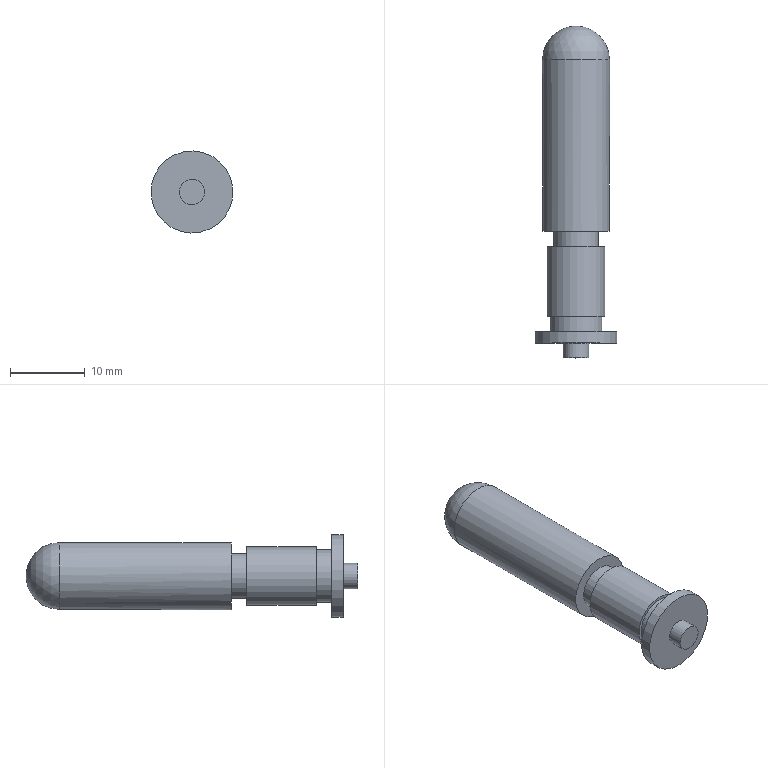Component | NX | VALVE_CORE | 1 solid | 13 faces | box 11 x 44.5 x 11 mm | volume 2399 mm3 | cylinder 6 | plane 6 | sphere 1 | commonest cylinder face diameters 11 x1 3.4 x1 7 x1 7.8 x1 6 x1 9 x1
STEP:
#1=CARTESIAN_POINT('',(0.,0.,0.));
#2=DIRECTION('',(0.,0.,1.));
#3=DIRECTION('',(1.,0.,0.));
#4=AXIS2_PLACEMENT_3D('',#1,#2,#3);
#5=CARTESIAN_POINT('',(9.389,-116.169,-3.008));
#6=VERTEX_POINT('',#5);
#7=CARTESIAN_POINT('',(13.994,-116.169,-0.));
#8=DIRECTION('',(0.,1.,0.));
#9=DIRECTION('',(-0.8372,0.,-0.5469));
#10=AXIS2_PLACEMENT_3D('',#7,#8,#9);
#11=CIRCLE('',#10,5.5);
#12=CARTESIAN_POINT('',(13.994,-116.169,-0.));
#13=DIRECTION('',(0.,-1.,0.));
#14=DIRECTION('',(-0.5469,0.,0.8372));
#15=AXIS2_PLACEMENT_3D('',#12,#13,#14);
#16=CYLINDRICAL_SURFACE('',#15,5.5);
#17=CARTESIAN_POINT('',(7.854,0.));
#18=DIRECTION('',(-1.,0.));
#19=VECTOR('',#18,1.);
#20=LINE('',#17,#19);
#21=(GEOMETRIC_REPRESENTATION_CONTEXT(2)PARAMETRIC_REPRESENTATION_CONTEXT()REPRESENTATION_CONTEXT('',''));
#22=DEFINITIONAL_REPRESENTATION('',(#20),#21);
#23=PCURVE('',#16,#22);
#24=CARTESIAN_POINT('',(13.994,-116.169,-0.));
#25=DIRECTION('',(0.,1.,0.));
#26=DIRECTION('',(0.5469,0.,-0.8372));
#27=AXIS2_PLACEMENT_3D('',#24,#25,#26);
#28=PLANE('',#27);
#29=CARTESIAN_POINT('',(0.,0.));
#30=DIRECTION('',(0.,1.));
#31=AXIS2_PLACEMENT_2D('',#29,#30);
#32=CIRCLE('',#31,5.5);
#33=(GEOMETRIC_REPRESENTATION_CONTEXT(2)PARAMETRIC_REPRESENTATION_CONTEXT()REPRESENTATION_CONTEXT('',''));
#34=DEFINITIONAL_REPRESENTATION('',(#32),#33);
#35=PCURVE('',#28,#34);
#36=SURFACE_CURVE('',#11,(#23,#35),.PCURVE_S1.);
#37=EDGE_CURVE('',#6,#6,#36,.T.);
#38=ORIENTED_EDGE('',*,*,#37,.F.);
#39=CARTESIAN_POINT('',(9.389,-117.669,-3.008));
#40=VERTEX_POINT('',#39);
#41=CARTESIAN_POINT('',(9.389,-116.169,-3.008));
#42=CARTESIAN_POINT('',(9.389,-117.669,-3.008));
#43=B_SPLINE_CURVE_WITH_KNOTS('',1,(#41,#42),.UNSPECIFIED.,.F.,.F.,(2,2),(0.,1.5),.PIECEWISE_BEZIER_KNOTS.);
#44=CARTESIAN_POINT('',(7.854,0.));
#45=DIRECTION('',(0.,1.));
#46=VECTOR('',#45,1.);
#47=LINE('',#44,#46);
#48=(GEOMETRIC_REPRESENTATION_CONTEXT(2)PARAMETRIC_REPRESENTATION_CONTEXT()REPRESENTATION_CONTEXT('',''));
#49=DEFINITIONAL_REPRESENTATION('',(#47),#48);
#50=PCURVE('',#16,#49);
#51=CARTESIAN_POINT('',(1.571,0.));
#52=DIRECTION('',(0.,1.));
#53=VECTOR('',#52,1.);
#54=LINE('',#51,#53);
#55=(GEOMETRIC_REPRESENTATION_CONTEXT(2)PARAMETRIC_REPRESENTATION_CONTEXT()REPRESENTATION_CONTEXT('',''));
#56=DEFINITIONAL_REPRESENTATION('',(#54),#55);
#57=PCURVE('',#16,#56);
#58=SEAM_CURVE('',#43,(#50,#57),.PCURVE_S1.);
#59=EDGE_CURVE('',#6,#40,#58,.T.);
#60=ORIENTED_EDGE('',*,*,#59,.T.);
#61=CARTESIAN_POINT('',(13.994,-117.669,-0.));
#62=DIRECTION('',(0.,1.,0.));
#63=DIRECTION('',(-0.8372,0.,-0.5469));
#64=AXIS2_PLACEMENT_3D('',#61,#62,#63);
#65=CIRCLE('',#64,5.5);
#66=CARTESIAN_POINT('',(7.854,1.5));
#67=DIRECTION('',(-1.,0.));
#68=VECTOR('',#67,1.);
#69=LINE('',#66,#68);
#70=(GEOMETRIC_REPRESENTATION_CONTEXT(2)PARAMETRIC_REPRESENTATION_CONTEXT()REPRESENTATION_CONTEXT('',''));
#71=DEFINITIONAL_REPRESENTATION('',(#69),#70);
#72=PCURVE('',#16,#71);
#73=CARTESIAN_POINT('',(13.994,-117.669,-0.));
#74=DIRECTION('',(0.,1.,0.));
#75=DIRECTION('',(0.5469,0.,-0.8372));
#76=AXIS2_PLACEMENT_3D('',#73,#74,#75);
#77=PLANE('',#76);
#78=CARTESIAN_POINT('',(0.,0.));
#79=DIRECTION('',(0.,1.));
#80=AXIS2_PLACEMENT_2D('',#78,#79);
#81=CIRCLE('',#80,5.5);
#82=(GEOMETRIC_REPRESENTATION_CONTEXT(2)PARAMETRIC_REPRESENTATION_CONTEXT()REPRESENTATION_CONTEXT('',''));
#83=DEFINITIONAL_REPRESENTATION('',(#81),#82);
#84=PCURVE('',#77,#83);
#85=SURFACE_CURVE('',#65,(#72,#84),.PCURVE_S1.);
#86=EDGE_CURVE('',#40,#40,#85,.T.);
#87=ORIENTED_EDGE('',*,*,#86,.T.);
#88=ORIENTED_EDGE('',*,*,#59,.F.);
#89=EDGE_LOOP('',(#38,#60,#87,#88));
#90=FACE_BOUND('',#89,.T.);
#91=ADVANCED_FACE('',(#90),#16,.T.);
#92=CARTESIAN_POINT('',(11.064,-116.169,-1.914));
#93=VERTEX_POINT('',#92);
#94=CARTESIAN_POINT('',(13.994,-116.169,-0.));
#95=DIRECTION('',(0.,1.,0.));
#96=DIRECTION('',(-0.8372,0.,-0.5469));
#97=AXIS2_PLACEMENT_3D('',#94,#95,#96);
#98=CIRCLE('',#97,3.5);
#99=CARTESIAN_POINT('',(0.,0.));
#100=DIRECTION('',(0.,1.));
#101=AXIS2_PLACEMENT_2D('',#99,#100);
#102=CIRCLE('',#101,3.5);
#103=(GEOMETRIC_REPRESENTATION_CONTEXT(2)PARAMETRIC_REPRESENTATION_CONTEXT()REPRESENTATION_CONTEXT('',''));
#104=DEFINITIONAL_REPRESENTATION('',(#102),#103);
#105=PCURVE('',#28,#104);
#106=CARTESIAN_POINT('',(13.994,-114.069,-0.));
#107=DIRECTION('',(0.,-1.,0.));
#108=DIRECTION('',(-0.5469,0.,0.8372));
#109=AXIS2_PLACEMENT_3D('',#106,#107,#108);
#110=CYLINDRICAL_SURFACE('',#109,3.5);
#111=CARTESIAN_POINT('',(7.854,2.1));
#112=DIRECTION('',(-1.,0.));
#113=VECTOR('',#112,1.);
#114=LINE('',#111,#113);
#115=(GEOMETRIC_REPRESENTATION_CONTEXT(2)PARAMETRIC_REPRESENTATION_CONTEXT()REPRESENTATION_CONTEXT('',''));
#116=DEFINITIONAL_REPRESENTATION('',(#114),#115);
#117=PCURVE('',#110,#116);
#118=SURFACE_CURVE('',#98,(#105,#117),.PCURVE_S1.);
#119=EDGE_CURVE('',#93,#93,#118,.T.);
#120=ORIENTED_EDGE('',*,*,#119,.F.);
#121=EDGE_LOOP('',(#120));
#122=FACE_BOUND('',#121,.T.);
#123=ORIENTED_EDGE('',*,*,#37,.T.);
#124=EDGE_LOOP('',(#123));
#125=FACE_BOUND('',#124,.T.);
#126=ADVANCED_FACE('',(#122,#125),#28,.T.);
#127=CARTESIAN_POINT('',(12.571,-117.669,-0.9298));
#128=VERTEX_POINT('',#127);
#129=CARTESIAN_POINT('',(13.994,-117.669,-0.));
#130=DIRECTION('',(0.,-1.,0.));
#131=DIRECTION('',(-0.8372,0.,-0.5469));
#132=AXIS2_PLACEMENT_3D('',#129,#130,#131);
#133=CIRCLE('',#132,1.7);
#134=CARTESIAN_POINT('',(0.,1.7));
#135=CARTESIAN_POINT('',(2.944,1.7));
#136=CARTESIAN_POINT('',(1.472,-0.85));
#137=CARTESIAN_POINT('',(0.,-3.4));
#138=CARTESIAN_POINT('',(-1.472,-0.85));
#139=CARTESIAN_POINT('',(-2.944,1.7));
#140=CARTESIAN_POINT('',(0.,1.7));
#141=(BOUNDED_CURVE()B_SPLINE_CURVE(2,(#134,#135,#136,#137,#138,#139,#140),.UNSPECIFIED.,.T.,.F.)B_SPLINE_CURVE_WITH_KNOTS((1,2,2,2,2,1),(-2.094,0.,2.094,4.189,6.283,8.378),.UNSPECIFIED.)CURVE()GEOMETRIC_REPRESENTATION_ITEM()RATIONAL_B_SPLINE_CURVE((1.,0.5,1.,0.5,1.,0.5,1.))REPRESENTATION_ITEM(''));
#142=(GEOMETRIC_REPRESENTATION_CONTEXT(2)PARAMETRIC_REPRESENTATION_CONTEXT()REPRESENTATION_CONTEXT('',''));
#143=DEFINITIONAL_REPRESENTATION('',(#141),#142);
#144=PCURVE('',#77,#143);
#145=CARTESIAN_POINT('',(13.994,-119.669,-0.));
#146=DIRECTION('',(0.,1.,0.));
#147=DIRECTION('',(0.5469,0.,-0.8372));
#148=AXIS2_PLACEMENT_3D('',#145,#146,#147);
#149=CYLINDRICAL_SURFACE('',#148,1.7);
#150=CARTESIAN_POINT('',(7.854,2.));
#151=DIRECTION('',(-1.,0.));
#152=VECTOR('',#151,1.);
#153=LINE('',#150,#152);
#154=(GEOMETRIC_REPRESENTATION_CONTEXT(2)PARAMETRIC_REPRESENTATION_CONTEXT()REPRESENTATION_CONTEXT('',''));
#155=DEFINITIONAL_REPRESENTATION('',(#153),#154);
#156=PCURVE('',#149,#155);
#157=SURFACE_CURVE('',#133,(#144,#156),.PCURVE_S1.);
#158=EDGE_CURVE('',#128,#128,#157,.T.);
#159=ORIENTED_EDGE('',*,*,#158,.F.);
#160=EDGE_LOOP('',(#159));
#161=FACE_BOUND('',#160,.T.);
#162=ORIENTED_EDGE('',*,*,#86,.F.);
#163=EDGE_LOOP('',(#162));
#164=FACE_BOUND('',#163,.T.);
#165=ADVANCED_FACE('',(#161,#164),#77,.F.);
#166=CARTESIAN_POINT('',(12.571,-119.669,-0.9298));
#167=VERTEX_POINT('',#166);
#168=CARTESIAN_POINT('',(13.994,-119.669,-0.));
#169=DIRECTION('',(0.,-1.,0.));
#170=DIRECTION('',(-0.8372,0.,-0.5469));
#171=AXIS2_PLACEMENT_3D('',#168,#169,#170);
#172=CIRCLE('',#171,1.7);
#173=CARTESIAN_POINT('',(7.854,0.));
#174=DIRECTION('',(-1.,0.));
#175=VECTOR('',#174,1.);
#176=LINE('',#173,#175);
#177=(GEOMETRIC_REPRESENTATION_CONTEXT(2)PARAMETRIC_REPRESENTATION_CONTEXT()REPRESENTATION_CONTEXT('',''));
#178=DEFINITIONAL_REPRESENTATION('',(#176),#177);
#179=PCURVE('',#149,#178);
#180=CARTESIAN_POINT('',(13.994,-119.669,-0.));
#181=DIRECTION('',(0.,-1.,0.));
#182=DIRECTION('',(-0.5469,0.,0.8372));
#183=AXIS2_PLACEMENT_3D('',#180,#181,#182);
#184=PLANE('',#183);
#185=CARTESIAN_POINT('',(0.,0.));
#186=DIRECTION('',(0.,1.));
#187=AXIS2_PLACEMENT_2D('',#185,#186);
#188=CIRCLE('',#187,1.7);
#189=(GEOMETRIC_REPRESENTATION_CONTEXT(2)PARAMETRIC_REPRESENTATION_CONTEXT()REPRESENTATION_CONTEXT('',''));
#190=DEFINITIONAL_REPRESENTATION('',(#188),#189);
#191=PCURVE('',#184,#190);
#192=SURFACE_CURVE('',#172,(#179,#191),.PCURVE_S1.);
#193=EDGE_CURVE('',#167,#167,#192,.T.);
#194=ORIENTED_EDGE('',*,*,#193,.F.);
#195=CARTESIAN_POINT('',(12.571,-119.669,-0.9298));
#196=CARTESIAN_POINT('',(12.571,-117.669,-0.9298));
#197=B_SPLINE_CURVE_WITH_KNOTS('',1,(#195,#196),.UNSPECIFIED.,.F.,.F.,(2,2),(0.,2.),.PIECEWISE_BEZIER_KNOTS.);
#198=CARTESIAN_POINT('',(7.854,0.));
#199=DIRECTION('',(0.,1.));
#200=VECTOR('',#199,1.);
#201=LINE('',#198,#200);
#202=(GEOMETRIC_REPRESENTATION_CONTEXT(2)PARAMETRIC_REPRESENTATION_CONTEXT()REPRESENTATION_CONTEXT('',''));
#203=DEFINITIONAL_REPRESENTATION('',(#201),#202);
#204=PCURVE('',#149,#203);
#205=CARTESIAN_POINT('',(1.571,0.));
#206=DIRECTION('',(0.,1.));
#207=VECTOR('',#206,1.);
#208=LINE('',#205,#207);
#209=(GEOMETRIC_REPRESENTATION_CONTEXT(2)PARAMETRIC_REPRESENTATION_CONTEXT()REPRESENTATION_CONTEXT('',''));
#210=DEFINITIONAL_REPRESENTATION('',(#208),#209);
#211=PCURVE('',#149,#210);
#212=SEAM_CURVE('',#197,(#204,#211),.PCURVE_S1.);
#213=EDGE_CURVE('',#167,#128,#212,.T.);
#214=ORIENTED_EDGE('',*,*,#213,.T.);
#215=ORIENTED_EDGE('',*,*,#158,.T.);
#216=ORIENTED_EDGE('',*,*,#213,.F.);
#217=EDGE_LOOP('',(#194,#214,#215,#216));
#218=FACE_BOUND('',#217,.T.);
#219=ADVANCED_FACE('',(#218),#149,.T.);
#220=ORIENTED_EDGE('',*,*,#193,.T.);
#221=EDGE_LOOP('',(#220));
#222=FACE_BOUND('',#221,.T.);
#223=ADVANCED_FACE('',(#222),#184,.T.);
#224=CARTESIAN_POINT('',(11.064,-114.069,-1.914));
#225=VERTEX_POINT('',#224);
#226=CARTESIAN_POINT('',(13.994,-114.069,-0.));
#227=DIRECTION('',(0.,1.,0.));
#228=DIRECTION('',(-0.8372,0.,-0.5469));
#229=AXIS2_PLACEMENT_3D('',#226,#227,#228);
#230=CIRCLE('',#229,3.5);
#231=CARTESIAN_POINT('',(7.854,0.));
#232=DIRECTION('',(-1.,0.));
#233=VECTOR('',#232,1.);
#234=LINE('',#231,#233);
#235=(GEOMETRIC_REPRESENTATION_CONTEXT(2)PARAMETRIC_REPRESENTATION_CONTEXT()REPRESENTATION_CONTEXT('',''));
#236=DEFINITIONAL_REPRESENTATION('',(#234),#235);
#237=PCURVE('',#110,#236);
#238=CARTESIAN_POINT('',(13.994,-114.069,-0.));
#239=DIRECTION('',(0.,1.,0.));
#240=DIRECTION('',(0.5469,0.,-0.8372));
#241=AXIS2_PLACEMENT_3D('',#238,#239,#240);
#242=PLANE('',#241);
#243=CARTESIAN_POINT('',(0.,0.));
#244=DIRECTION('',(0.,1.));
#245=AXIS2_PLACEMENT_2D('',#243,#244);
#246=CIRCLE('',#245,3.5);
#247=(GEOMETRIC_REPRESENTATION_CONTEXT(2)PARAMETRIC_REPRESENTATION_CONTEXT()REPRESENTATION_CONTEXT('',''));
#248=DEFINITIONAL_REPRESENTATION('',(#246),#247);
#249=PCURVE('',#242,#248);
#250=SURFACE_CURVE('',#230,(#237,#249),.PCURVE_S1.);
#251=EDGE_CURVE('',#225,#225,#250,.T.);
#252=ORIENTED_EDGE('',*,*,#251,.F.);
#253=CARTESIAN_POINT('',(11.064,-114.069,-1.914));
#254=CARTESIAN_POINT('',(11.064,-116.169,-1.914));
#255=B_SPLINE_CURVE_WITH_KNOTS('',1,(#253,#254),.UNSPECIFIED.,.F.,.F.,(2,2),(0.,2.1),.PIECEWISE_BEZIER_KNOTS.);
#256=CARTESIAN_POINT('',(7.854,0.));
#257=DIRECTION('',(0.,1.));
#258=VECTOR('',#257,1.);
#259=LINE('',#256,#258);
#260=(GEOMETRIC_REPRESENTATION_CONTEXT(2)PARAMETRIC_REPRESENTATION_CONTEXT()REPRESENTATION_CONTEXT('',''));
#261=DEFINITIONAL_REPRESENTATION('',(#259),#260);
#262=PCURVE('',#110,#261);
#263=CARTESIAN_POINT('',(1.571,0.));
#264=DIRECTION('',(0.,1.));
#265=VECTOR('',#264,1.);
#266=LINE('',#263,#265);
#267=(GEOMETRIC_REPRESENTATION_CONTEXT(2)PARAMETRIC_REPRESENTATION_CONTEXT()REPRESENTATION_CONTEXT('',''));
#268=DEFINITIONAL_REPRESENTATION('',(#266),#267);
#269=PCURVE('',#110,#268);
#270=SEAM_CURVE('',#255,(#262,#269),.PCURVE_S1.);
#271=EDGE_CURVE('',#225,#93,#270,.T.);
#272=ORIENTED_EDGE('',*,*,#271,.T.);
#273=ORIENTED_EDGE('',*,*,#119,.T.);
#274=ORIENTED_EDGE('',*,*,#271,.F.);
#275=EDGE_LOOP('',(#252,#272,#273,#274));
#276=FACE_BOUND('',#275,.T.);
#277=ADVANCED_FACE('',(#276),#110,.T.);
#278=CARTESIAN_POINT('',(10.729,-104.769,-2.133));
#279=VERTEX_POINT('',#278);
#280=CARTESIAN_POINT('',(13.994,-104.769,-0.));
#281=DIRECTION('',(0.,1.,0.));
#282=DIRECTION('',(-0.8372,0.,-0.5469));
#283=AXIS2_PLACEMENT_3D('',#280,#281,#282);
#284=CIRCLE('',#283,3.9);
#285=CARTESIAN_POINT('',(13.994,-104.769,-0.));
#286=DIRECTION('',(0.,-1.,0.));
#287=DIRECTION('',(-0.5469,0.,0.8372));
#288=AXIS2_PLACEMENT_3D('',#285,#286,#287);
#289=CYLINDRICAL_SURFACE('',#288,3.9);
#290=CARTESIAN_POINT('',(7.854,0.));
#291=DIRECTION('',(-1.,0.));
#292=VECTOR('',#291,1.);
#293=LINE('',#290,#292);
#294=(GEOMETRIC_REPRESENTATION_CONTEXT(2)PARAMETRIC_REPRESENTATION_CONTEXT()REPRESENTATION_CONTEXT('',''));
#295=DEFINITIONAL_REPRESENTATION('',(#293),#294);
#296=PCURVE('',#289,#295);
#297=CARTESIAN_POINT('',(13.994,-104.769,-0.));
#298=DIRECTION('',(0.,1.,0.));
#299=DIRECTION('',(0.5469,0.,-0.8372));
#300=AXIS2_PLACEMENT_3D('',#297,#298,#299);
#301=PLANE('',#300);
#302=CARTESIAN_POINT('',(0.,0.));
#303=DIRECTION('',(0.,1.));
#304=AXIS2_PLACEMENT_2D('',#302,#303);
#305=CIRCLE('',#304,3.9);
#306=(GEOMETRIC_REPRESENTATION_CONTEXT(2)PARAMETRIC_REPRESENTATION_CONTEXT()REPRESENTATION_CONTEXT('',''));
#307=DEFINITIONAL_REPRESENTATION('',(#305),#306);
#308=PCURVE('',#301,#307);
#309=SURFACE_CURVE('',#284,(#296,#308),.PCURVE_S1.);
#310=EDGE_CURVE('',#279,#279,#309,.T.);
#311=ORIENTED_EDGE('',*,*,#310,.F.);
#312=CARTESIAN_POINT('',(10.729,-114.069,-2.133));
#313=VERTEX_POINT('',#312);
#314=CARTESIAN_POINT('',(10.729,-104.769,-2.133));
#315=CARTESIAN_POINT('',(10.729,-114.069,-2.133));
#316=B_SPLINE_CURVE_WITH_KNOTS('',1,(#314,#315),.UNSPECIFIED.,.F.,.F.,(2,2),(0.,9.3),.PIECEWISE_BEZIER_KNOTS.);
#317=CARTESIAN_POINT('',(7.854,0.));
#318=DIRECTION('',(0.,1.));
#319=VECTOR('',#318,1.);
#320=LINE('',#317,#319);
#321=(GEOMETRIC_REPRESENTATION_CONTEXT(2)PARAMETRIC_REPRESENTATION_CONTEXT()REPRESENTATION_CONTEXT('',''));
#322=DEFINITIONAL_REPRESENTATION('',(#320),#321);
#323=PCURVE('',#289,#322);
#324=CARTESIAN_POINT('',(1.571,0.));
#325=DIRECTION('',(0.,1.));
#326=VECTOR('',#325,1.);
#327=LINE('',#324,#326);
#328=(GEOMETRIC_REPRESENTATION_CONTEXT(2)PARAMETRIC_REPRESENTATION_CONTEXT()REPRESENTATION_CONTEXT('',''));
#329=DEFINITIONAL_REPRESENTATION('',(#327),#328);
#330=PCURVE('',#289,#329);
#331=SEAM_CURVE('',#316,(#323,#330),.PCURVE_S1.);
#332=EDGE_CURVE('',#279,#313,#331,.T.);
#333=ORIENTED_EDGE('',*,*,#332,.T.);
#334=CARTESIAN_POINT('',(13.994,-114.069,-0.));
#335=DIRECTION('',(0.,1.,0.));
#336=DIRECTION('',(-0.8372,0.,-0.5469));
#337=AXIS2_PLACEMENT_3D('',#334,#335,#336);
#338=CIRCLE('',#337,3.9);
#339=CARTESIAN_POINT('',(7.854,9.3));
#340=DIRECTION('',(-1.,0.));
#341=VECTOR('',#340,1.);
#342=LINE('',#339,#341);
#343=(GEOMETRIC_REPRESENTATION_CONTEXT(2)PARAMETRIC_REPRESENTATION_CONTEXT()REPRESENTATION_CONTEXT('',''));
#344=DEFINITIONAL_REPRESENTATION('',(#342),#343);
#345=PCURVE('',#289,#344);
#346=CARTESIAN_POINT('',(0.,0.));
#347=DIRECTION('',(0.,1.));
#348=AXIS2_PLACEMENT_2D('',#346,#347);
#349=CIRCLE('',#348,3.9);
#350=(GEOMETRIC_REPRESENTATION_CONTEXT(2)PARAMETRIC_REPRESENTATION_CONTEXT()REPRESENTATION_CONTEXT('',''));
#351=DEFINITIONAL_REPRESENTATION('',(#349),#350);
#352=PCURVE('',#242,#351);
#353=SURFACE_CURVE('',#338,(#345,#352),.PCURVE_S1.);
#354=EDGE_CURVE('',#313,#313,#353,.T.);
#355=ORIENTED_EDGE('',*,*,#354,.T.);
#356=ORIENTED_EDGE('',*,*,#332,.F.);
#357=EDGE_LOOP('',(#311,#333,#355,#356));
#358=FACE_BOUND('',#357,.T.);
#359=ADVANCED_FACE('',(#358),#289,.T.);
#360=CARTESIAN_POINT('',(11.482,-104.769,-1.641));
#361=VERTEX_POINT('',#360);
#362=CARTESIAN_POINT('',(13.994,-104.769,-0.));
#363=DIRECTION('',(0.,1.,0.));
#364=DIRECTION('',(-0.8372,0.,-0.5469));
#365=AXIS2_PLACEMENT_3D('',#362,#363,#364);
#366=CIRCLE('',#365,3.);
#367=CARTESIAN_POINT('',(0.,0.));
#368=DIRECTION('',(0.,1.));
#369=AXIS2_PLACEMENT_2D('',#367,#368);
#370=CIRCLE('',#369,3.);
#371=(GEOMETRIC_REPRESENTATION_CONTEXT(2)PARAMETRIC_REPRESENTATION_CONTEXT()REPRESENTATION_CONTEXT('',''));
#372=DEFINITIONAL_REPRESENTATION('',(#370),#371);
#373=PCURVE('',#301,#372);
#374=CARTESIAN_POINT('',(13.994,-102.669,-0.));
#375=DIRECTION('',(0.,-1.,0.));
#376=DIRECTION('',(-0.5469,0.,0.8372));
#377=AXIS2_PLACEMENT_3D('',#374,#375,#376);
#378=CYLINDRICAL_SURFACE('',#377,3.);
#379=CARTESIAN_POINT('',(7.854,2.1));
#380=DIRECTION('',(-1.,0.));
#381=VECTOR('',#380,1.);
#382=LINE('',#379,#381);
#383=(GEOMETRIC_REPRESENTATION_CONTEXT(2)PARAMETRIC_REPRESENTATION_CONTEXT()REPRESENTATION_CONTEXT('',''));
#384=DEFINITIONAL_REPRESENTATION('',(#382),#383);
#385=PCURVE('',#378,#384);
#386=SURFACE_CURVE('',#366,(#373,#385),.PCURVE_S1.);
#387=EDGE_CURVE('',#361,#361,#386,.T.);
#388=ORIENTED_EDGE('',*,*,#387,.F.);
#389=EDGE_LOOP('',(#388));
#390=FACE_BOUND('',#389,.T.);
#391=ORIENTED_EDGE('',*,*,#310,.T.);
#392=EDGE_LOOP('',(#391));
#393=FACE_BOUND('',#392,.T.);
#394=ADVANCED_FACE('',(#390,#393),#301,.T.);
#395=ORIENTED_EDGE('',*,*,#251,.T.);
#396=EDGE_LOOP('',(#395));
#397=FACE_BOUND('',#396,.T.);
#398=ORIENTED_EDGE('',*,*,#354,.F.);
#399=EDGE_LOOP('',(#398));
#400=FACE_BOUND('',#399,.T.);
#401=ADVANCED_FACE('',(#397,#400),#242,.F.);
#402=CARTESIAN_POINT('',(11.482,-102.669,-1.641));
#403=VERTEX_POINT('',#402);
#404=CARTESIAN_POINT('',(13.994,-102.669,-0.));
#405=DIRECTION('',(0.,1.,0.));
#406=DIRECTION('',(-0.8372,0.,-0.5469));
#407=AXIS2_PLACEMENT_3D('',#404,#405,#406);
#408=CIRCLE('',#407,3.);
#409=CARTESIAN_POINT('',(7.854,0.));
#410=DIRECTION('',(-1.,0.));
#411=VECTOR('',#410,1.);
#412=LINE('',#409,#411);
#413=(GEOMETRIC_REPRESENTATION_CONTEXT(2)PARAMETRIC_REPRESENTATION_CONTEXT()REPRESENTATION_CONTEXT('',''));
#414=DEFINITIONAL_REPRESENTATION('',(#412),#413);
#415=PCURVE('',#378,#414);
#416=CARTESIAN_POINT('',(13.994,-102.669,-0.));
#417=DIRECTION('',(0.,1.,0.));
#418=DIRECTION('',(0.5469,0.,-0.8372));
#419=AXIS2_PLACEMENT_3D('',#416,#417,#418);
#420=PLANE('',#419);
#421=CARTESIAN_POINT('',(0.,0.));
#422=DIRECTION('',(0.,1.));
#423=AXIS2_PLACEMENT_2D('',#421,#422);
#424=CIRCLE('',#423,3.);
#425=(GEOMETRIC_REPRESENTATION_CONTEXT(2)PARAMETRIC_REPRESENTATION_CONTEXT()REPRESENTATION_CONTEXT('',''));
#426=DEFINITIONAL_REPRESENTATION('',(#424),#425);
#427=PCURVE('',#420,#426);
#428=SURFACE_CURVE('',#408,(#415,#427),.PCURVE_S1.);
#429=EDGE_CURVE('',#403,#403,#428,.T.);
#430=ORIENTED_EDGE('',*,*,#429,.F.);
#431=CARTESIAN_POINT('',(11.482,-102.669,-1.641));
#432=CARTESIAN_POINT('',(11.482,-104.769,-1.641));
#433=B_SPLINE_CURVE_WITH_KNOTS('',1,(#431,#432),.UNSPECIFIED.,.F.,.F.,(2,2),(0.,2.1),.PIECEWISE_BEZIER_KNOTS.);
#434=CARTESIAN_POINT('',(7.854,0.));
#435=DIRECTION('',(0.,1.));
#436=VECTOR('',#435,1.);
#437=LINE('',#434,#436);
#438=(GEOMETRIC_REPRESENTATION_CONTEXT(2)PARAMETRIC_REPRESENTATION_CONTEXT()REPRESENTATION_CONTEXT('',''));
#439=DEFINITIONAL_REPRESENTATION('',(#437),#438);
#440=PCURVE('',#378,#439);
#441=CARTESIAN_POINT('',(1.571,0.));
#442=DIRECTION('',(0.,1.));
#443=VECTOR('',#442,1.);
#444=LINE('',#441,#443);
#445=(GEOMETRIC_REPRESENTATION_CONTEXT(2)PARAMETRIC_REPRESENTATION_CONTEXT()REPRESENTATION_CONTEXT('',''));
#446=DEFINITIONAL_REPRESENTATION('',(#444),#445);
#447=PCURVE('',#378,#446);
#448=SEAM_CURVE('',#433,(#440,#447),.PCURVE_S1.);
#449=EDGE_CURVE('',#403,#361,#448,.T.);
#450=ORIENTED_EDGE('',*,*,#449,.T.);
#451=ORIENTED_EDGE('',*,*,#387,.T.);
#452=ORIENTED_EDGE('',*,*,#449,.F.);
#453=EDGE_LOOP('',(#430,#450,#451,#452));
#454=FACE_BOUND('',#453,.T.);
#455=ADVANCED_FACE('',(#454),#378,.T.);
#456=CARTESIAN_POINT('',(11.533,-79.669,3.767));
#457=VERTEX_POINT('',#456);
#458=CARTESIAN_POINT('',(16.455,-79.669,-3.767));
#459=VERTEX_POINT('',#458);
#460=CARTESIAN_POINT('',(13.994,-79.669,-0.));
#461=DIRECTION('',(0.,-1.,0.));
#462=DIRECTION('',(-0.5469,0.,0.8372));
#463=AXIS2_PLACEMENT_3D('',#460,#461,#462);
#464=CIRCLE('',#463,4.5);
#465=CARTESIAN_POINT('',(13.994,-75.169,-0.));
#466=DIRECTION('',(0.,-1.,0.));
#467=DIRECTION('',(-0.5469,0.,0.8372));
#468=AXIS2_PLACEMENT_3D('',#465,#466,#467);
#469=CYLINDRICAL_SURFACE('',#468,4.5);
#470=CARTESIAN_POINT('',(0.,4.5));
#471=DIRECTION('',(1.,0.));
#472=VECTOR('',#471,1.);
#473=LINE('',#470,#472);
#474=(GEOMETRIC_REPRESENTATION_CONTEXT(2)PARAMETRIC_REPRESENTATION_CONTEXT()REPRESENTATION_CONTEXT('',''));
#475=DEFINITIONAL_REPRESENTATION('',(#473),#474);
#476=PCURVE('',#469,#475);
#477=CARTESIAN_POINT('',(13.994,-79.669,-0.));
#478=DIRECTION('',(0.,1.,-0.));
#479=DIRECTION('',(0.5469,-0.,-0.8372));
#480=AXIS2_PLACEMENT_3D('',#477,#478,#479);
#481=SPHERICAL_SURFACE('',#480,4.5);
#482=CARTESIAN_POINT('',(3.142,0.));
#483=CARTESIAN_POINT('',(3.046,0.));
#484=CARTESIAN_POINT('',(2.856,0.));
#485=CARTESIAN_POINT('',(2.57,0.));
#486=CARTESIAN_POINT('',(2.285,0.));
#487=CARTESIAN_POINT('',(1.999,0.));
#488=CARTESIAN_POINT('',(1.714,0.));
#489=CARTESIAN_POINT('',(1.428,0.));
#490=CARTESIAN_POINT('',(1.142,0.));
#491=CARTESIAN_POINT('',(0.8568,0.));
#492=CARTESIAN_POINT('',(0.5712,0.));
#493=CARTESIAN_POINT('',(0.2856,0.));
#494=CARTESIAN_POINT('',(0.,0.));
#495=CARTESIAN_POINT('',(-0.2856,0.));
#496=CARTESIAN_POINT('',(-0.5712,0.));
#497=CARTESIAN_POINT('',(-0.8568,0.));
#498=CARTESIAN_POINT('',(-1.142,0.));
#499=CARTESIAN_POINT('',(-1.428,0.));
#500=CARTESIAN_POINT('',(-1.714,0.));
#501=CARTESIAN_POINT('',(-1.999,0.));
#502=CARTESIAN_POINT('',(-2.285,0.));
#503=CARTESIAN_POINT('',(-2.57,0.));
#504=CARTESIAN_POINT('',(-2.856,0.));
#505=CARTESIAN_POINT('',(-3.046,0.));
#506=CARTESIAN_POINT('',(-3.142,0.));
#507=B_SPLINE_CURVE_WITH_KNOTS('',3,(#482,#483,#484,#485,#486,#487,#488,#489,#490,#491,#492,#493,#494,#495,#496,#497,#498,#499,#500,#501,#502,#503,#504,#505,#506),.UNSPECIFIED.,.F.,.F.,(4,1,1,1,1,1,1,1,1,1,1,1,1,1,1,1,1,1,1,1,1,1,4),(0.,0.2856,0.5712,0.8568,1.142,1.428,1.714,1.999,2.285,2.57,2.856,3.142,3.427,3.713,3.998,4.284,4.57,4.855,5.141,5.426,5.712,5.998,6.283),.QUASI_UNIFORM_KNOTS.);
#508=(GEOMETRIC_REPRESENTATION_CONTEXT(2)PARAMETRIC_REPRESENTATION_CONTEXT()REPRESENTATION_CONTEXT('',''));
#509=DEFINITIONAL_REPRESENTATION('',(#507),#508);
#510=PCURVE('',#481,#509);
#511=SURFACE_CURVE('',#464,(#476,#510),.PCURVE_S1.);
#512=EDGE_CURVE('',#457,#459,#511,.T.);
#513=ORIENTED_EDGE('',*,*,#512,.T.);
#514=CARTESIAN_POINT('',(13.994,-79.669,-0.));
#515=DIRECTION('',(0.,-1.,0.));
#516=DIRECTION('',(-0.5469,0.,0.8372));
#517=AXIS2_PLACEMENT_3D('',#514,#515,#516);
#518=CIRCLE('',#517,4.5);
#519=CARTESIAN_POINT('',(0.,4.5));
#520=DIRECTION('',(1.,0.));
#521=VECTOR('',#520,1.);
#522=LINE('',#519,#521);
#523=(GEOMETRIC_REPRESENTATION_CONTEXT(2)PARAMETRIC_REPRESENTATION_CONTEXT()REPRESENTATION_CONTEXT('',''));
#524=DEFINITIONAL_REPRESENTATION('',(#522),#523);
#525=PCURVE('',#469,#524);
#526=CARTESIAN_POINT('',(9.425,0.));
#527=CARTESIAN_POINT('',(9.33,0.));
#528=CARTESIAN_POINT('',(9.139,0.));
#529=CARTESIAN_POINT('',(8.854,0.));
#530=CARTESIAN_POINT('',(8.568,0.));
#531=CARTESIAN_POINT('',(8.282,0.));
#532=CARTESIAN_POINT('',(7.997,0.));
#533=CARTESIAN_POINT('',(7.711,0.));
#534=CARTESIAN_POINT('',(7.426,0.));
#535=CARTESIAN_POINT('',(7.14,0.));
#536=CARTESIAN_POINT('',(6.854,0.));
#537=CARTESIAN_POINT('',(6.569,0.));
#538=CARTESIAN_POINT('',(6.283,0.));
#539=CARTESIAN_POINT('',(5.998,0.));
#540=CARTESIAN_POINT('',(5.712,0.));
#541=CARTESIAN_POINT('',(5.426,0.));
#542=CARTESIAN_POINT('',(5.141,0.));
#543=CARTESIAN_POINT('',(4.855,0.));
#544=CARTESIAN_POINT('',(4.57,0.));
#545=CARTESIAN_POINT('',(4.284,0.));
#546=CARTESIAN_POINT('',(3.998,0.));
#547=CARTESIAN_POINT('',(3.713,0.));
#548=CARTESIAN_POINT('',(3.427,0.));
#549=CARTESIAN_POINT('',(3.237,0.));
#550=CARTESIAN_POINT('',(3.142,0.));
#551=B_SPLINE_CURVE_WITH_KNOTS('',3,(#526,#527,#528,#529,#530,#531,#532,#533,#534,#535,#536,#537,#538,#539,#540,#541,#542,#543,#544,#545,#546,#547,#548,#549,#550),.UNSPECIFIED.,.F.,.F.,(4,1,1,1,1,1,1,1,1,1,1,1,1,1,1,1,1,1,1,1,1,1,4),(0.,0.2856,0.5712,0.8568,1.142,1.428,1.714,1.999,2.285,2.57,2.856,3.142,3.427,3.713,3.998,4.284,4.57,4.855,5.141,5.426,5.712,5.998,6.283),.QUASI_UNIFORM_KNOTS.);
#552=(GEOMETRIC_REPRESENTATION_CONTEXT(2)PARAMETRIC_REPRESENTATION_CONTEXT()REPRESENTATION_CONTEXT('',''));
#553=DEFINITIONAL_REPRESENTATION('',(#551),#552);
#554=PCURVE('',#481,#553);
#555=SURFACE_CURVE('',#518,(#525,#554),.PCURVE_S1.);
#556=EDGE_CURVE('',#459,#457,#555,.T.);
#557=ORIENTED_EDGE('',*,*,#556,.T.);
#558=CARTESIAN_POINT('',(11.533,-102.669,3.767));
#559=VERTEX_POINT('',#558);
#560=CARTESIAN_POINT('',(11.533,-79.669,3.767));
#561=CARTESIAN_POINT('',(11.533,-102.669,3.767));
#562=B_SPLINE_CURVE_WITH_KNOTS('',1,(#560,#561),.UNSPECIFIED.,.F.,.F.,(2,2),(4.5,27.5),.PIECEWISE_BEZIER_KNOTS.);
#563=CARTESIAN_POINT('',(6.283,0.));
#564=DIRECTION('',(0.,1.));
#565=VECTOR('',#564,1.);
#566=LINE('',#563,#565);
#567=(GEOMETRIC_REPRESENTATION_CONTEXT(2)PARAMETRIC_REPRESENTATION_CONTEXT()REPRESENTATION_CONTEXT('',''));
#568=DEFINITIONAL_REPRESENTATION('',(#566),#567);
#569=PCURVE('',#469,#568);
#570=CARTESIAN_POINT('',(0.,0.));
#571=DIRECTION('',(0.,1.));
#572=VECTOR('',#571,1.);
#573=LINE('',#570,#572);
#574=(GEOMETRIC_REPRESENTATION_CONTEXT(2)PARAMETRIC_REPRESENTATION_CONTEXT()REPRESENTATION_CONTEXT('',''));
#575=DEFINITIONAL_REPRESENTATION('',(#573),#574);
#576=PCURVE('',#469,#575);
#577=SEAM_CURVE('',#562,(#569,#576),.PCURVE_S1.);
#578=EDGE_CURVE('',#457,#559,#577,.T.);
#579=ORIENTED_EDGE('',*,*,#578,.T.);
#580=CARTESIAN_POINT('',(10.227,-102.669,-2.461));
#581=VERTEX_POINT('',#580);
#582=CARTESIAN_POINT('',(13.994,-102.669,-0.));
#583=DIRECTION('',(0.,1.,0.));
#584=DIRECTION('',(-0.8372,0.,-0.5469));
#585=AXIS2_PLACEMENT_3D('',#582,#583,#584);
#586=CIRCLE('',#585,4.5);
#587=CARTESIAN_POINT('',(7.854,27.5));
#588=DIRECTION('',(-1.,0.));
#589=VECTOR('',#588,1.);
#590=LINE('',#587,#589);
#591=(GEOMETRIC_REPRESENTATION_CONTEXT(2)PARAMETRIC_REPRESENTATION_CONTEXT()REPRESENTATION_CONTEXT('',''));
#592=DEFINITIONAL_REPRESENTATION('',(#590),#591);
#593=PCURVE('',#469,#592);
#594=CARTESIAN_POINT('',(0.,0.));
#595=DIRECTION('',(0.,1.));
#596=AXIS2_PLACEMENT_2D('',#594,#595);
#597=CIRCLE('',#596,4.5);
#598=(GEOMETRIC_REPRESENTATION_CONTEXT(2)PARAMETRIC_REPRESENTATION_CONTEXT()REPRESENTATION_CONTEXT('',''));
#599=DEFINITIONAL_REPRESENTATION('',(#597),#598);
#600=PCURVE('',#420,#599);
#601=SURFACE_CURVE('',#586,(#593,#600),.PCURVE_S1.);
#602=EDGE_CURVE('',#559,#581,#601,.T.);
#603=ORIENTED_EDGE('',*,*,#602,.T.);
#604=CARTESIAN_POINT('',(13.994,-102.669,-0.));
#605=DIRECTION('',(0.,1.,0.));
#606=DIRECTION('',(-0.8372,0.,-0.5469));
#607=AXIS2_PLACEMENT_3D('',#604,#605,#606);
#608=CIRCLE('',#607,4.5);
#609=CARTESIAN_POINT('',(1.571,27.5));
#610=DIRECTION('',(-1.,0.));
#611=VECTOR('',#610,1.);
#612=LINE('',#609,#611);
#613=(GEOMETRIC_REPRESENTATION_CONTEXT(2)PARAMETRIC_REPRESENTATION_CONTEXT()REPRESENTATION_CONTEXT('',''));
#614=DEFINITIONAL_REPRESENTATION('',(#612),#613);
#615=PCURVE('',#469,#614);
#616=CARTESIAN_POINT('',(0.,0.));
#617=DIRECTION('',(0.,1.));
#618=AXIS2_PLACEMENT_2D('',#616,#617);
#619=CIRCLE('',#618,4.5);
#620=(GEOMETRIC_REPRESENTATION_CONTEXT(2)PARAMETRIC_REPRESENTATION_CONTEXT()REPRESENTATION_CONTEXT('',''));
#621=DEFINITIONAL_REPRESENTATION('',(#619),#620);
#622=PCURVE('',#420,#621);
#623=SURFACE_CURVE('',#608,(#615,#622),.PCURVE_S1.);
#624=EDGE_CURVE('',#581,#559,#623,.T.);
#625=ORIENTED_EDGE('',*,*,#624,.T.);
#626=ORIENTED_EDGE('',*,*,#578,.F.);
#627=EDGE_LOOP('',(#513,#557,#579,#603,#625,#626));
#628=FACE_BOUND('',#627,.T.);
#629=ADVANCED_FACE('',(#628),#469,.T.);
#630=ORIENTED_EDGE('',*,*,#429,.T.);
#631=EDGE_LOOP('',(#630));
#632=FACE_BOUND('',#631,.T.);
#633=ORIENTED_EDGE('',*,*,#624,.F.);
#634=ORIENTED_EDGE('',*,*,#602,.F.);
#635=EDGE_LOOP('',(#633,#634));
#636=FACE_BOUND('',#635,.T.);
#637=ADVANCED_FACE('',(#632,#636),#420,.F.);
#638=ORIENTED_EDGE('',*,*,#556,.F.);
#639=CARTESIAN_POINT('',(13.994,-75.169,-0.));
#640=VERTEX_POINT('',#639);
#641=CARTESIAN_POINT('',(16.455,-79.669,-3.767));
#642=CARTESIAN_POINT('',(16.455,-78.491,-3.767));
#643=CARTESIAN_POINT('',(16.253,-77.313,-3.457));
#644=CARTESIAN_POINT('',(15.848,-76.28,-2.837));
#645=CARTESIAN_POINT('',(15.283,-75.539,-1.972));
#646=CARTESIAN_POINT('',(14.638,-75.169,-0.9863));
#647=CARTESIAN_POINT('',(13.994,-75.169,-0.));
#648=B_SPLINE_CURVE_WITH_KNOTS('',6,(#641,#642,#643,#644,#645,#646,#647),.UNSPECIFIED.,.F.,.F.,(7,7),(0.,1.571),.PIECEWISE_BEZIER_KNOTS.);
#649=CARTESIAN_POINT('',(6.283,0.));
#650=DIRECTION('',(0.,1.));
#651=VECTOR('',#650,1.);
#652=LINE('',#649,#651);
#653=(GEOMETRIC_REPRESENTATION_CONTEXT(2)PARAMETRIC_REPRESENTATION_CONTEXT()REPRESENTATION_CONTEXT('',''));
#654=DEFINITIONAL_REPRESENTATION('',(#652),#653);
#655=PCURVE('',#481,#654);
#656=CARTESIAN_POINT('',(0.,0.));
#657=DIRECTION('',(0.,1.));
#658=VECTOR('',#657,1.);
#659=LINE('',#656,#658);
#660=(GEOMETRIC_REPRESENTATION_CONTEXT(2)PARAMETRIC_REPRESENTATION_CONTEXT()REPRESENTATION_CONTEXT('',''));
#661=DEFINITIONAL_REPRESENTATION('',(#659),#660);
#662=PCURVE('',#481,#661);
#663=SEAM_CURVE('',#648,(#655,#662),.PCURVE_S1.);
#664=EDGE_CURVE('',#459,#640,#663,.T.);
#665=ORIENTED_EDGE('',*,*,#664,.T.);
#666=ORIENTED_EDGE('',*,*,#664,.F.);
#667=ORIENTED_EDGE('',*,*,#512,.F.);
#668=EDGE_LOOP('',(#638,#665,#666,#667));
#669=FACE_BOUND('',#668,.T.);
#670=ADVANCED_FACE('',(#669),#481,.T.);
#671=CLOSED_SHELL('',(#91,#126,#165,#219,#223,#277,#359,#394,#401,#455,#629,#637,#670));
#672=MANIFOLD_SOLID_BREP('',#671);
#673=(LENGTH_UNIT()NAMED_UNIT(*)SI_UNIT(.MILLI.,.METRE.));
#674=UNCERTAINTY_MEASURE_WITH_UNIT(LENGTH_MEASURE(0.00001),#673,'','');
#675=(NAMED_UNIT(*)PLANE_ANGLE_UNIT()SI_UNIT($,.RADIAN.));
#676=(NAMED_UNIT(*)SI_UNIT($,.STERADIAN.)SOLID_ANGLE_UNIT());
#677=(GEOMETRIC_REPRESENTATION_CONTEXT(3)GLOBAL_UNCERTAINTY_ASSIGNED_CONTEXT((#674))GLOBAL_UNIT_ASSIGNED_CONTEXT((#673,#675,#676))REPRESENTATION_CONTEXT('',''));
#678=ADVANCED_BREP_SHAPE_REPRESENTATION('',(#4,#672),#677);